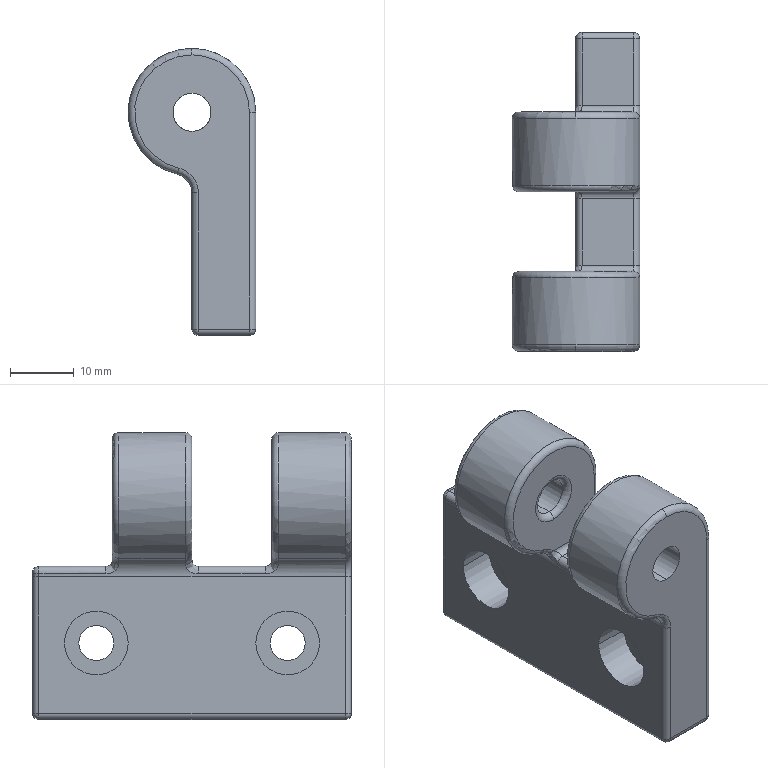Component | SolidWorks | FrameAssembly-1_Hinge-1-1_Hinge-1 | 1 solid | 75 faces | volume 18755 mm3 | cylinder 34 | torus 20 | plane 12 | sphere 6 | spline 3 | commonest cylinder face diameters 2 x19 6 x5 5.5 x4 10 x4 20 x2